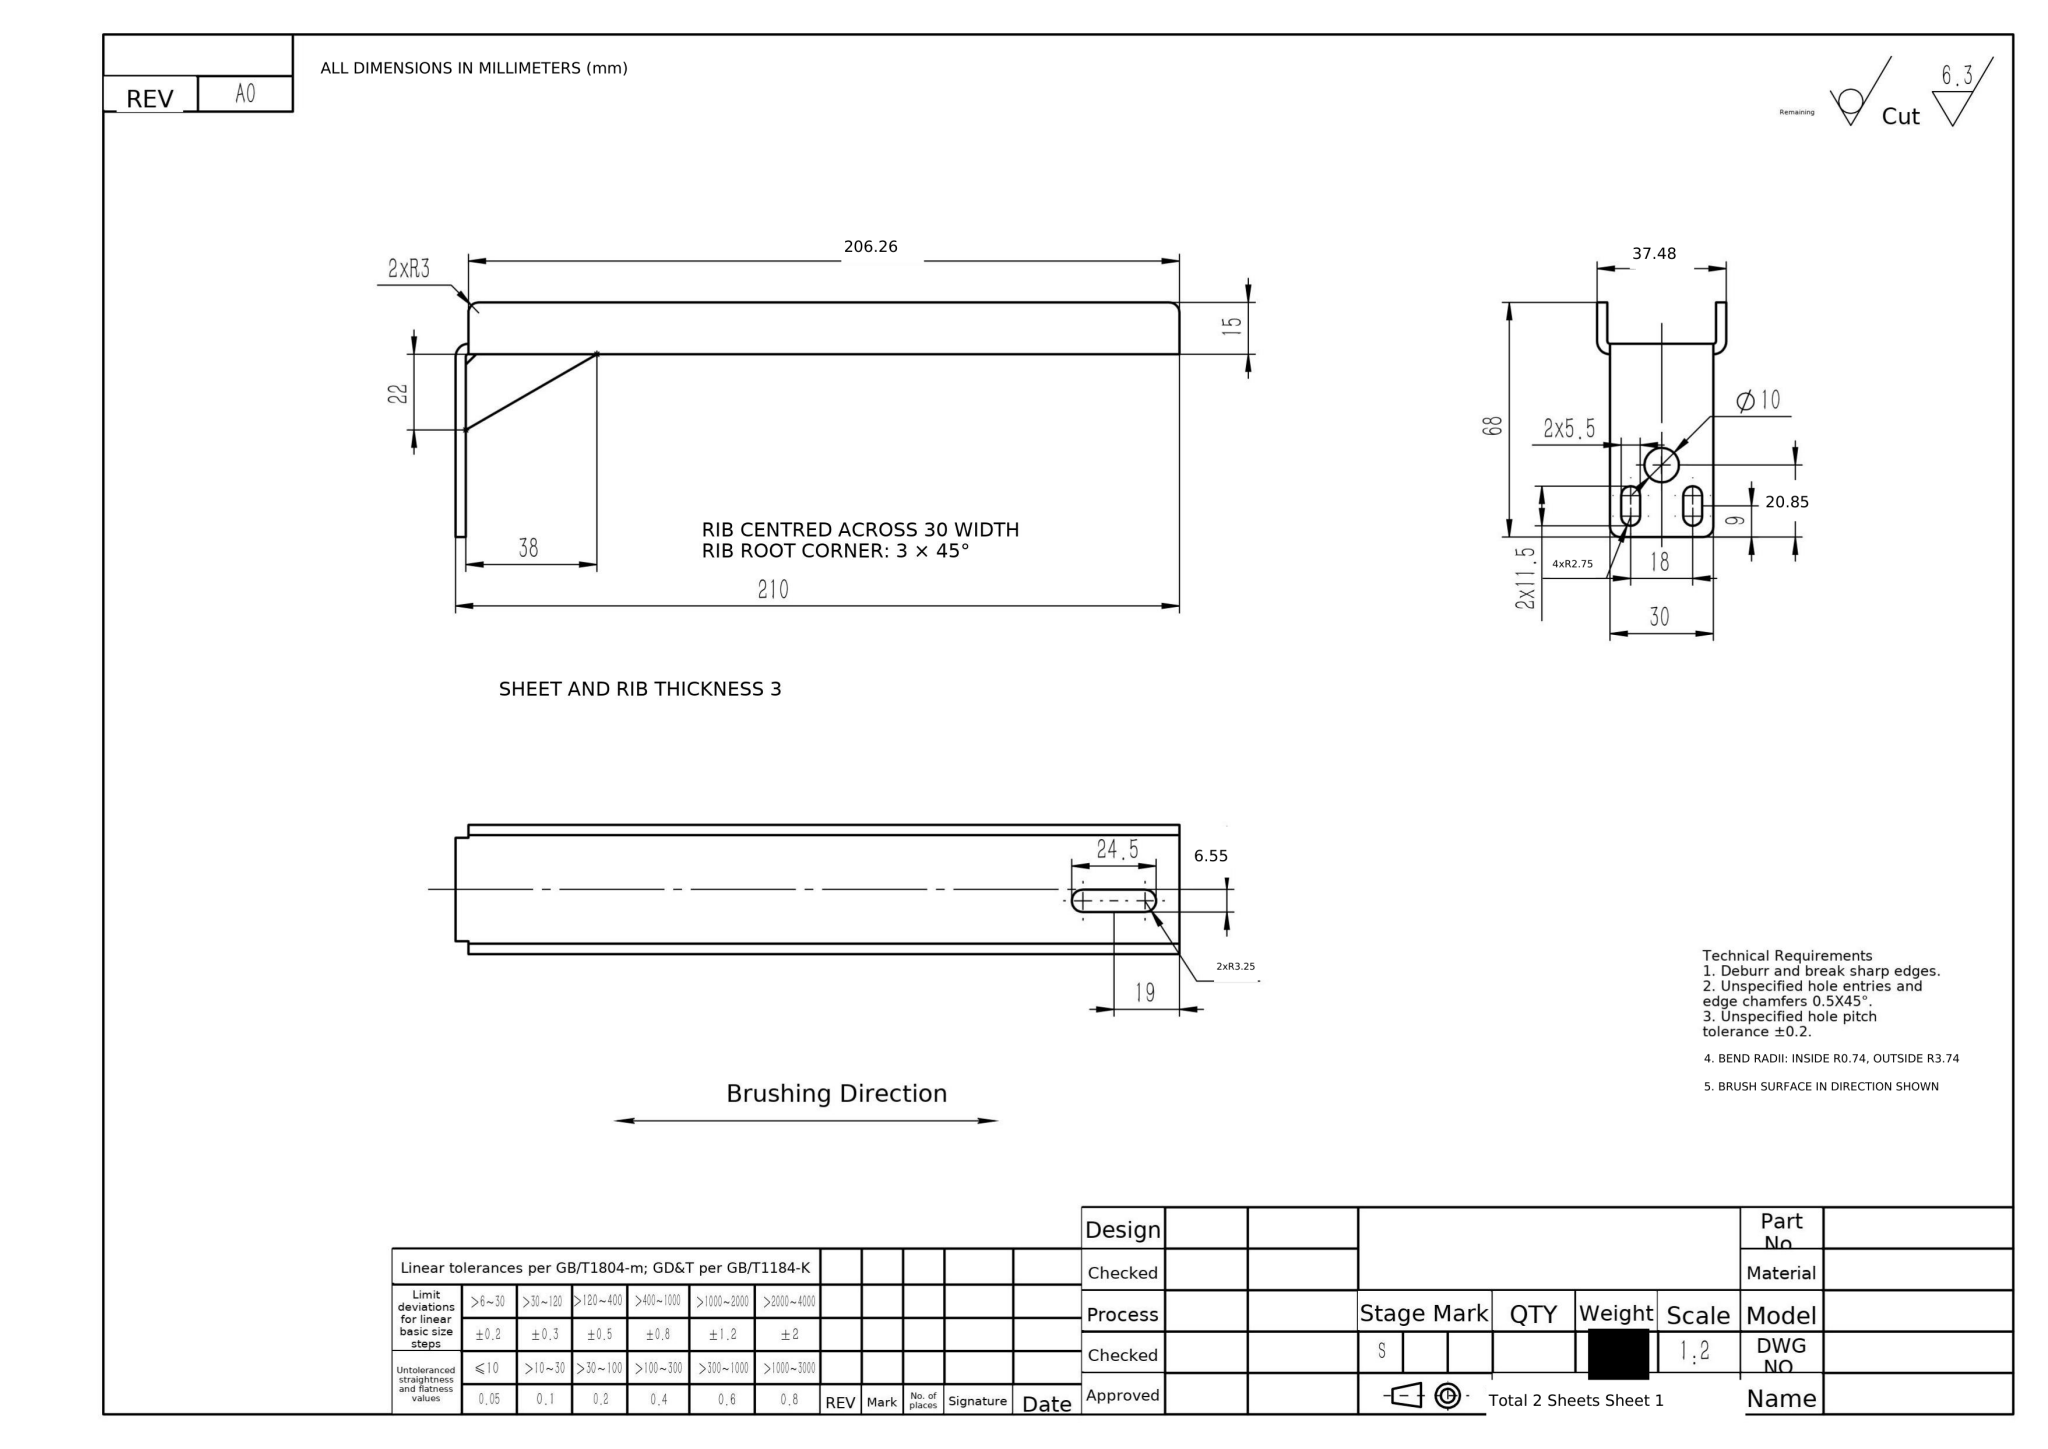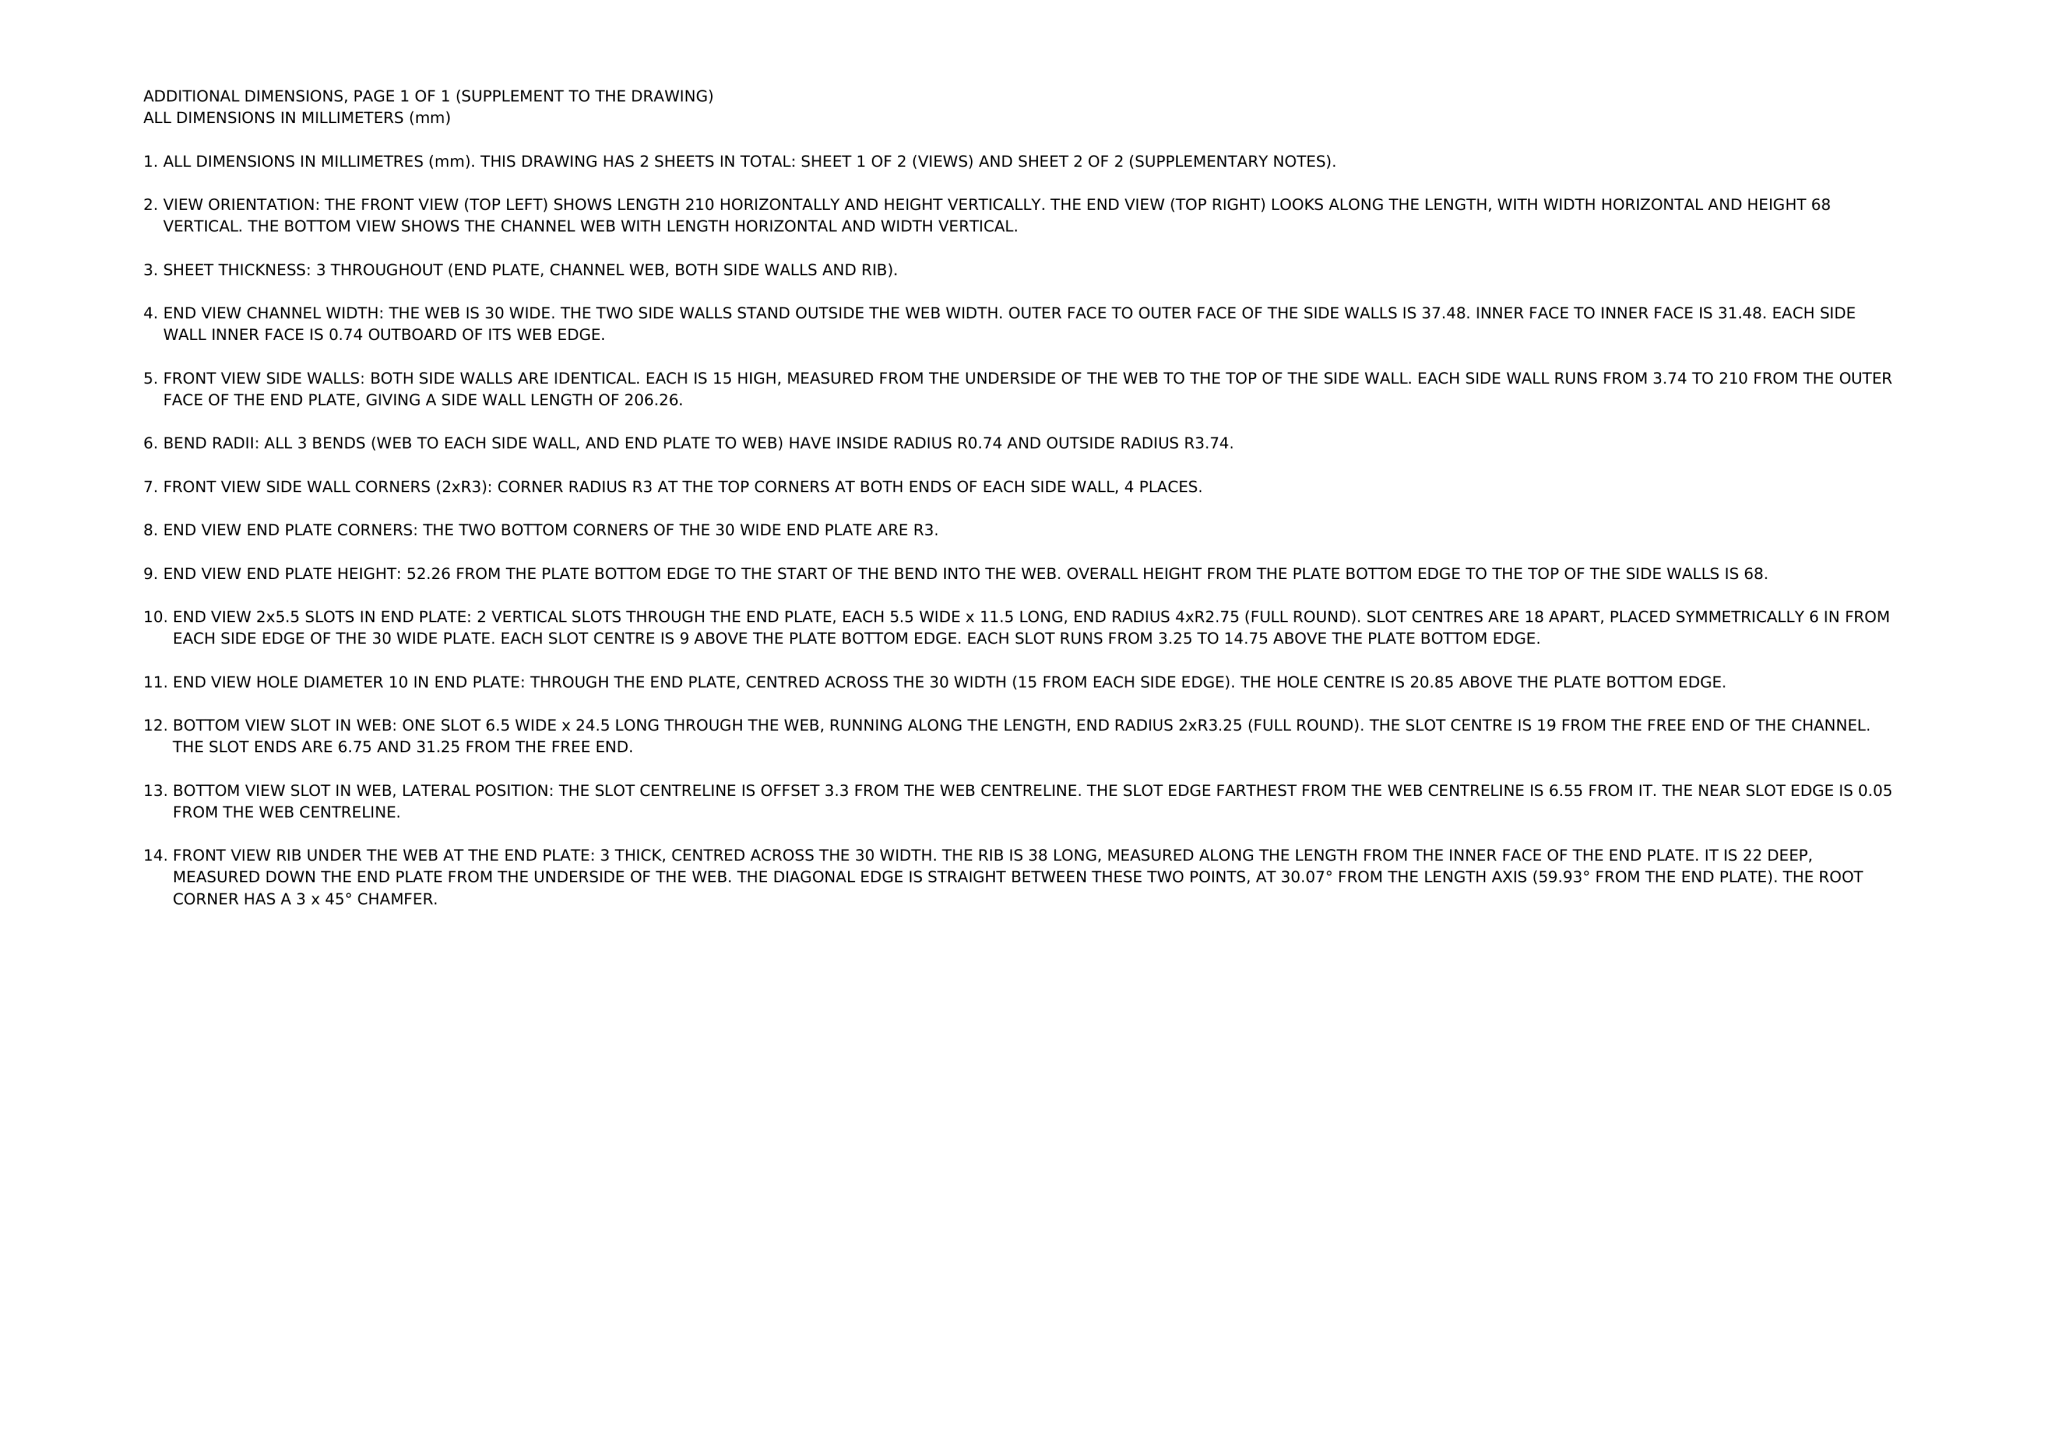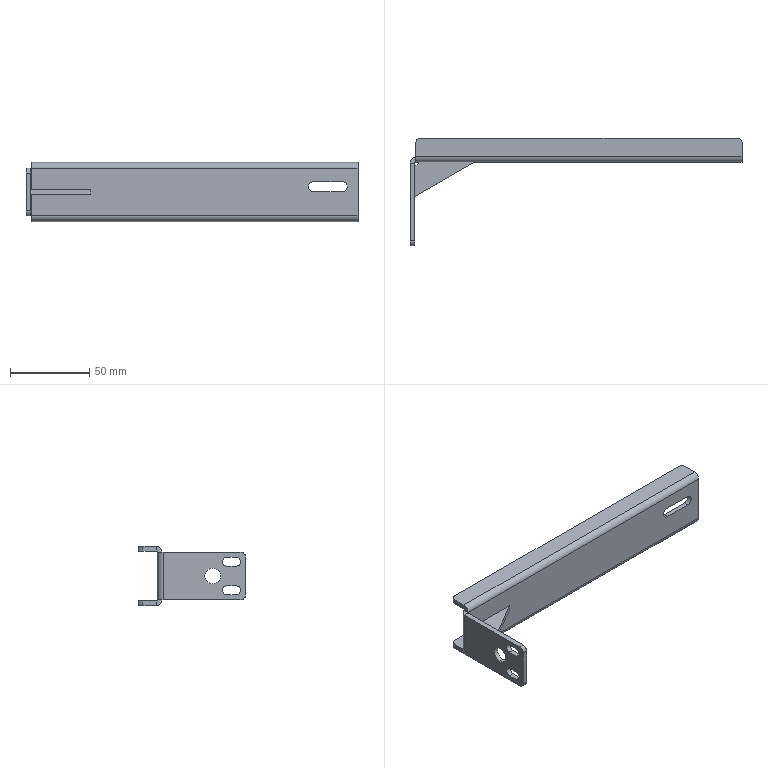Part | NX | mm | 1 solid | 54 faces | box 210 x 68 x 37.47 mm | volume 42050 mm3 | plane 34 | cylinder 20 | commonest cylinder face diameters 6 x6 5.5 x4 7.473 x3 1.473 x3 10 x2 6.5 x2